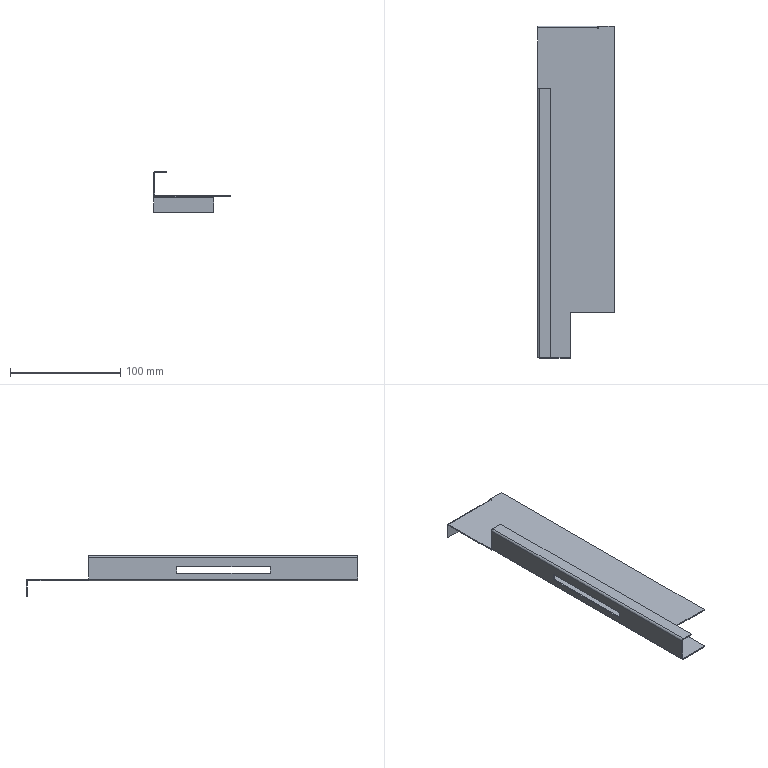Component | SolidWorks | CCQ-1.1-5SideUpperPlate3-2 | 1 solid | 46 faces | volume 27294 mm3 | plane 40 | cylinder 6 | commonest cylinder face diameters 3.473 x3 1.473 x3 | material 304